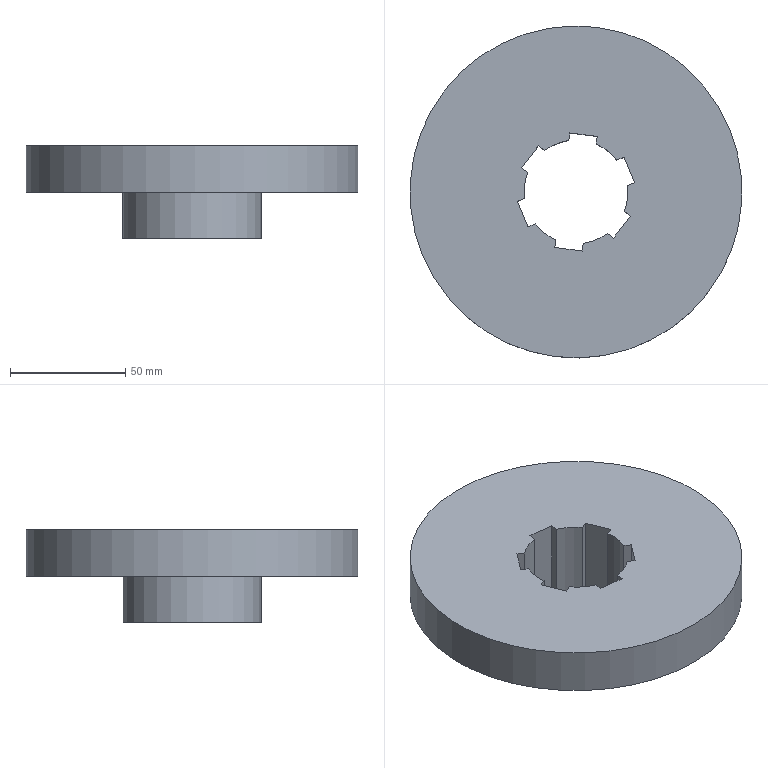Component | NX | ZHOUV3 | 1 solid | 29 faces | volume 309519 mm3 | plane 21 | cylinder 8 | commonest cylinder face diameters 45 x6 143.75 x1 60 x1